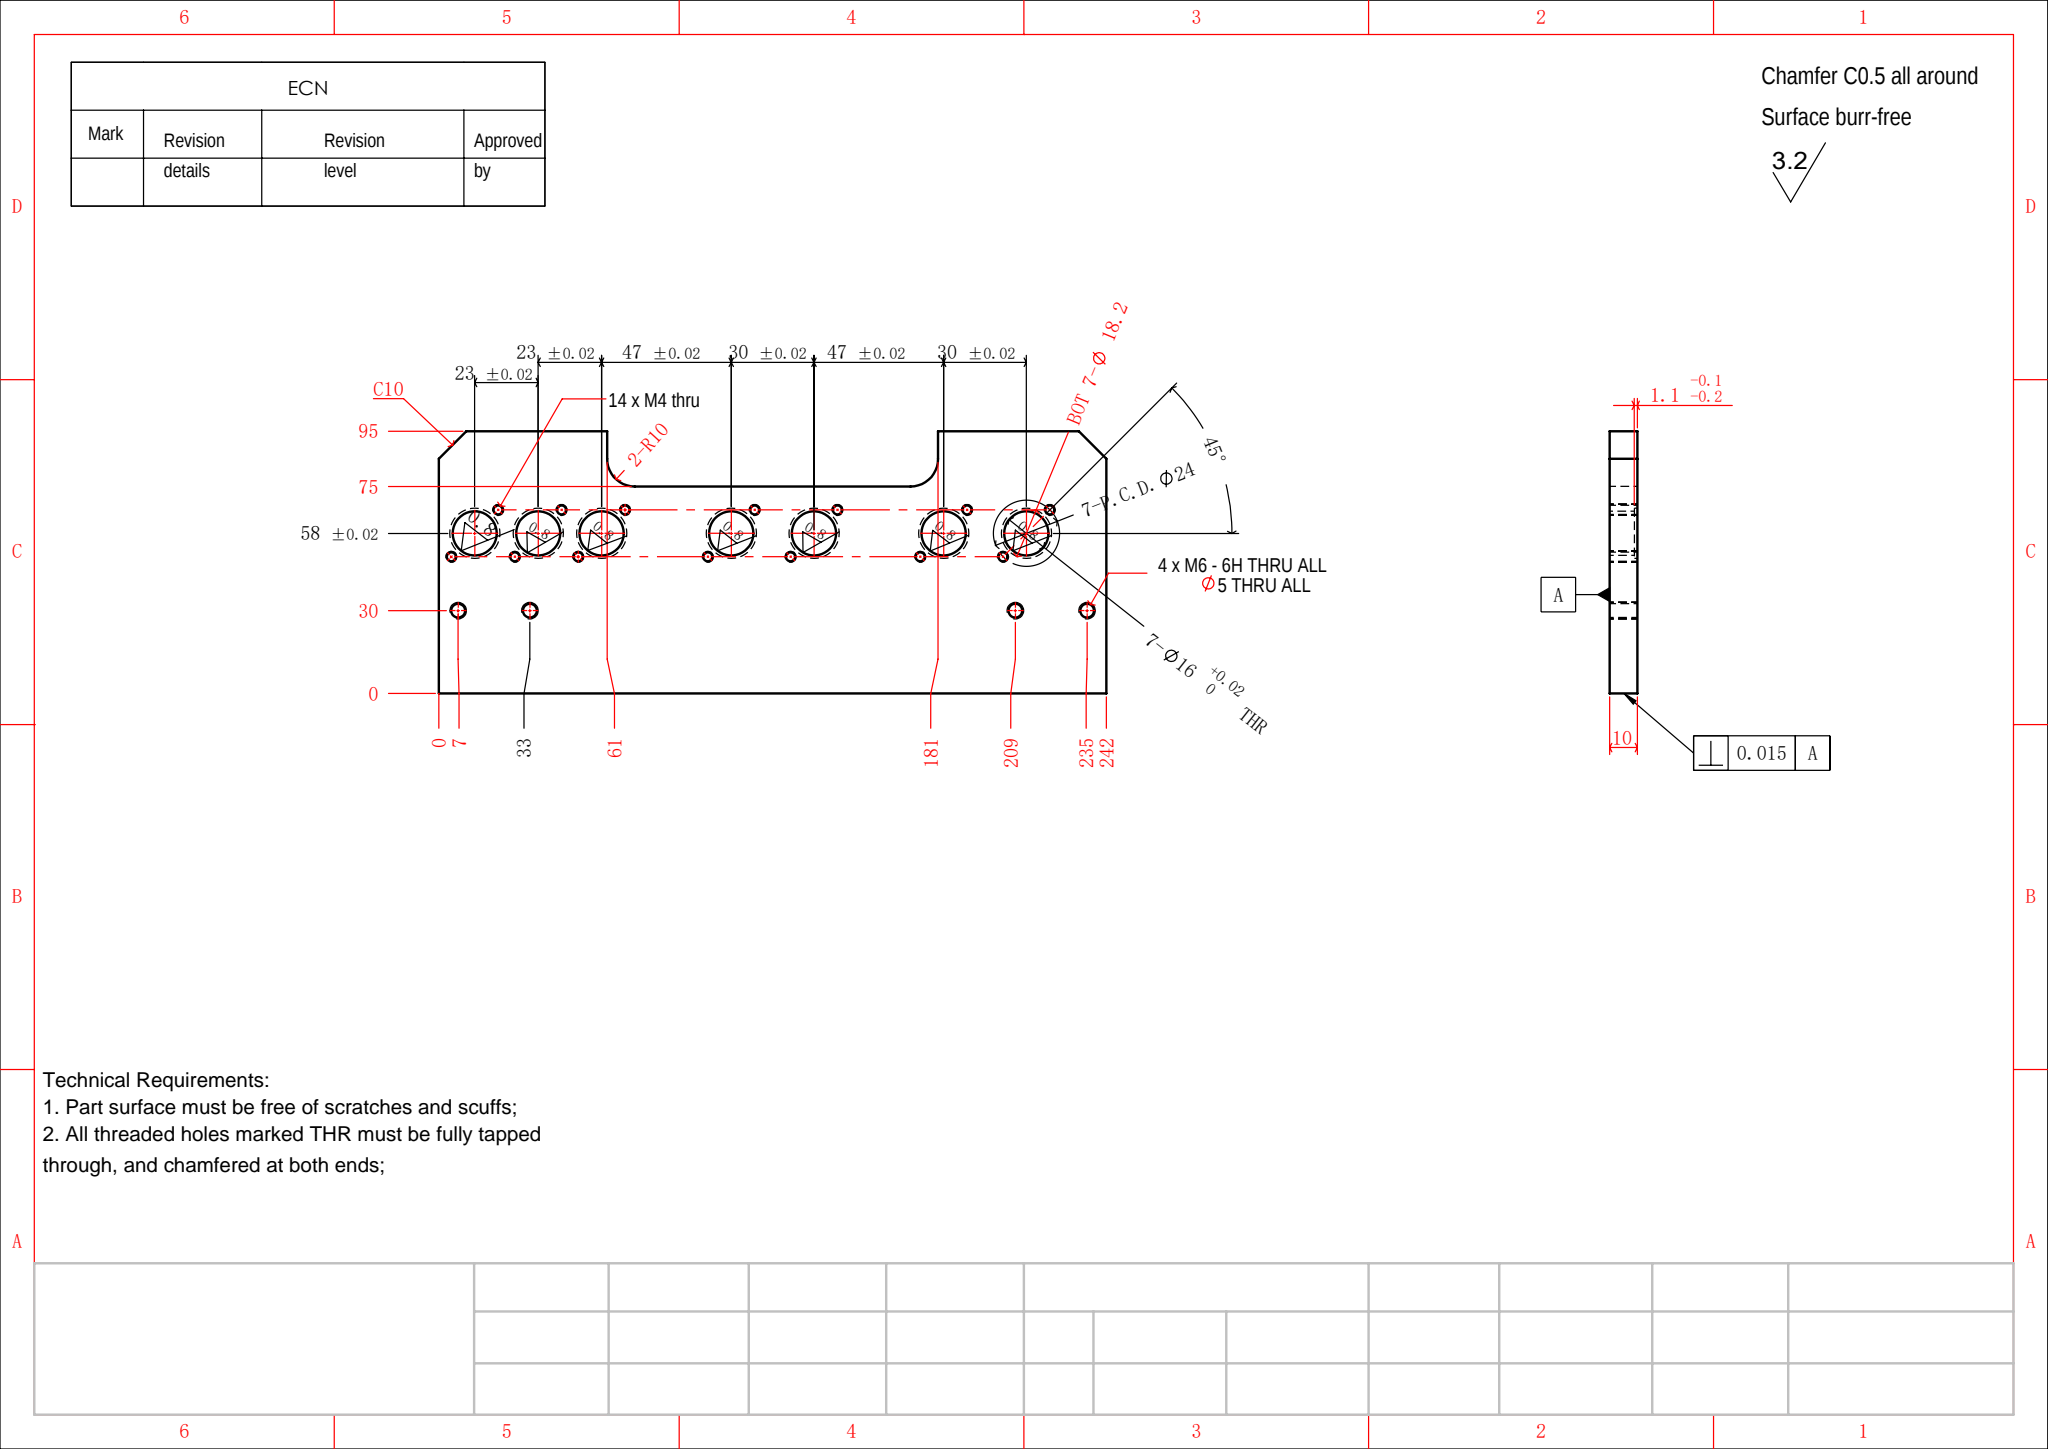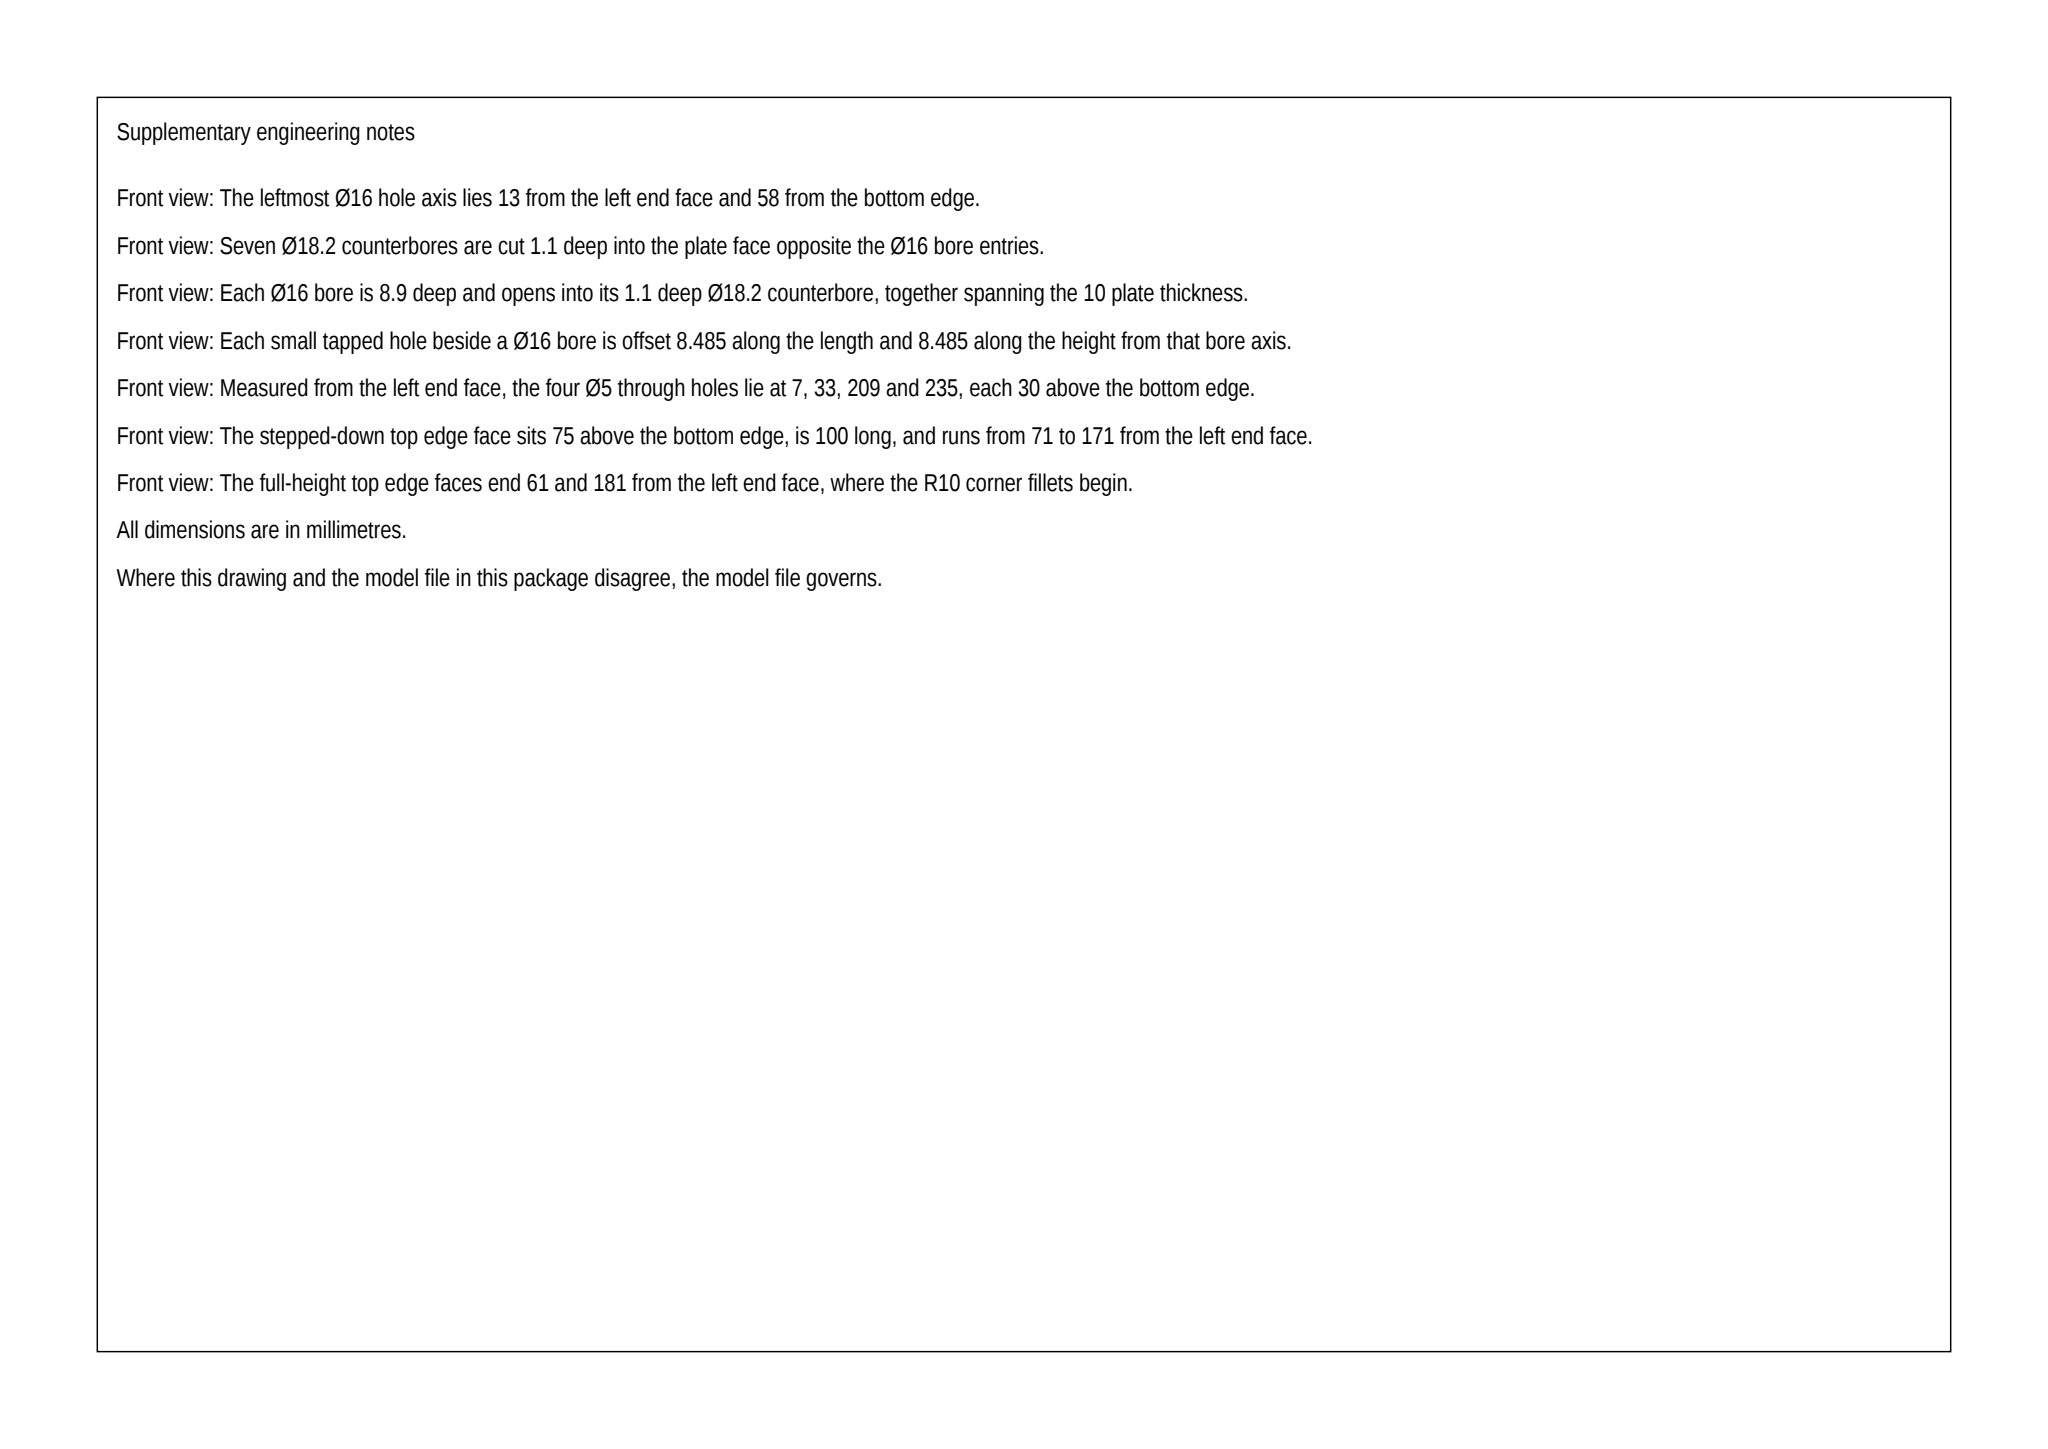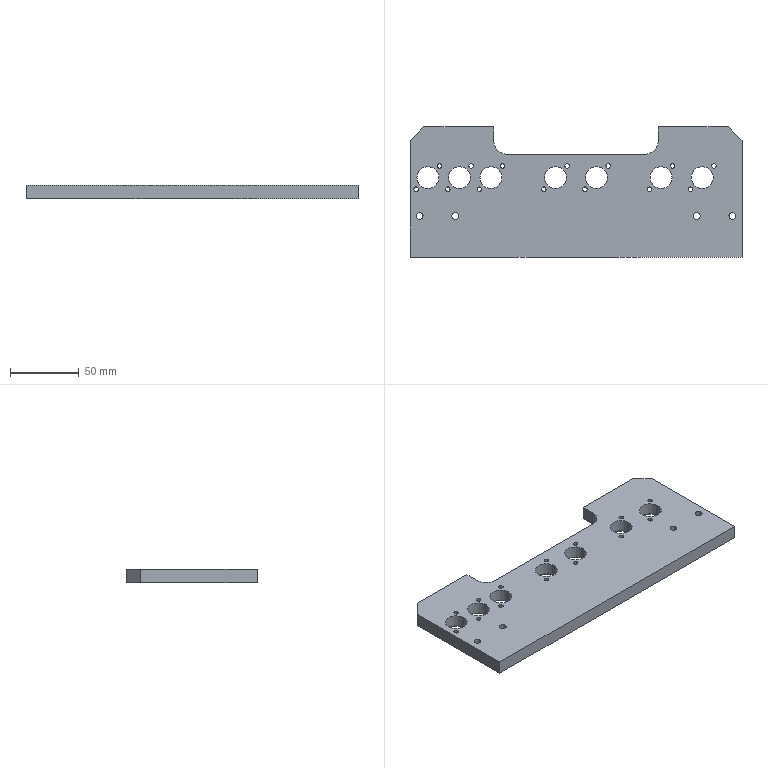Part | SolidWorks | mm | 1 solid | 85 faces | box 242 x 95 x 10 mm | volume 188817 mm3 | cylinder 66 | plane 19 | commonest cylinder face diameters 3.3 x28 18.2 x14 16 x14 5 x8 20 x2
Drawing notes:
OVERALL PLATE 242 LG x 95 HI x 10 THK | from the solid: bbox_xyz [242.0, 95.0, 10.0]; x-planes 0 & 242, y-planes 0 & 95, z-planes 0 & 10
TOP CUTOUT 120 W x 20 DP, SIDES AT 61 & 181 FROM LH EDGE, R10 CNRS | from the solid: x-planes 61 & 181; y-planes 75 & 95; Ø20 cyls (R10) at (71,85) and (171,85)
BOT FACE: 7X CBORE Ø18.2 DP 1.1 COAX W/ Ø16 THR HOLES | from the solid: Ø18.2 cyls len 1.1 at x=13,36,59,106,136,183,213 y=58; z-plane 1.1 x7; Ø16 len 8.9 same CL
7-Ø16 PATTERN: 13 FROM LH EDGE TO 1ST HOLE, 29 TO RH EDGE | from the solid: Ø16 holes at x=13,36,59,106,136,183,213; bbox x=0..242 -> 13 and 242-213=29